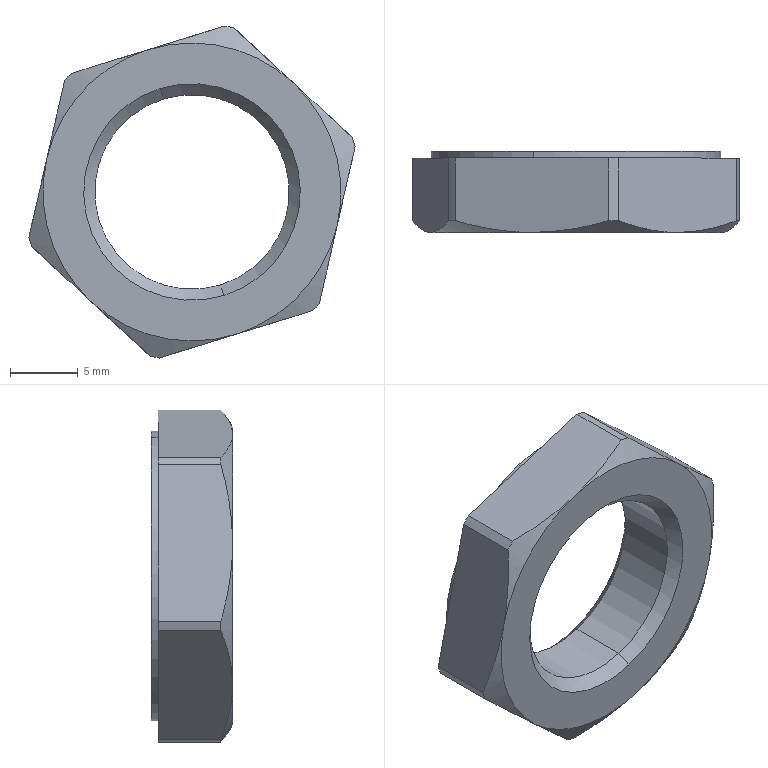Component | SolidWorks | gbgb16 MA NutF8-1 | 1 solid | 29 faces | box 24.09 x 6 x 24.52 mm | volume 1467 mm3 | cone 10 | cylinder 10 | plane 9 | commonest cylinder face diameters 25 x6 14.376 x2 21.4 x2
STEP:
#1=CARTESIAN_POINT('',(3.084,19.257,17.209));
#2=VERTEX_POINT('',#1);
#3=CARTESIAN_POINT('',(3.251,19.257,16.668));
#4=VERTEX_POINT('',#3);
#5=CARTESIAN_POINT('',(3.167,19.257,16.938));
#6=DIRECTION('',(0.,-1.,-0.));
#7=DIRECTION('',(0.2949,0.,-0.9555));
#8=AXIS2_PLACEMENT_3D('',#5,#6,#7);
#9=CIRCLE('',#8,0.283);
#10=EDGE_CURVE('',#2,#4,#9,.T.);
#11=ORIENTED_EDGE('',*,*,#10,.T.);
#12=CARTESIAN_POINT('',(3.26,19.289,16.637));
#13=VERTEX_POINT('',#12);
#14=CARTESIAN_POINT('',(3.26,19.289,16.637));
#15=DIRECTION('',(0.2085,0.7071,-0.6757));
#16=VECTOR('',#15,39.37);
#17=LINE('',#14,#16);
#18=EDGE_CURVE('',#4,#13,#17,.T.);
#19=ORIENTED_EDGE('',*,*,#18,.T.);
#20=CARTESIAN_POINT('',(3.074,19.289,17.239));
#21=VERTEX_POINT('',#20);
#22=CARTESIAN_POINT('',(3.167,19.289,16.938));
#23=DIRECTION('',(0.,-1.,-0.));
#24=DIRECTION('',(0.2949,0.,-0.9555));
#25=AXIS2_PLACEMENT_3D('',#22,#23,#24);
#26=CIRCLE('',#25,0.315);
#27=EDGE_CURVE('',#21,#13,#26,.T.);
#28=ORIENTED_EDGE('',*,*,#27,.F.);
#29=CARTESIAN_POINT('',(3.074,19.289,17.239));
#30=DIRECTION('',(-0.2085,0.7071,0.6757));
#31=VECTOR('',#30,39.37);
#32=LINE('',#29,#31);
#33=EDGE_CURVE('',#2,#21,#32,.T.);
#34=ORIENTED_EDGE('',*,*,#33,.F.);
#35=EDGE_LOOP('',(#11,#19,#28,#34));
#36=FACE_OUTER_BOUND('',#35,.T.);
#37=CARTESIAN_POINT('',(3.167,19.289,16.938));
#38=DIRECTION('',(-0.,1.,0.));
#39=DIRECTION('',(-0.2949,-0.,0.9555));
#40=AXIS2_PLACEMENT_3D('',#37,#38,#39);
#41=CONICAL_SURFACE('',#40,0.315,0.7854);
#42=ADVANCED_FACE('',(#36),#41,.F.);
#43=ORIENTED_EDGE('',*,*,#10,.F.);
#44=CARTESIAN_POINT('',(3.084,19.085,17.209));
#45=VERTEX_POINT('',#44);
#46=CARTESIAN_POINT('',(3.084,19.289,17.209));
#47=DIRECTION('',(0.,-1.,-0.));
#48=VECTOR('',#47,39.37);
#49=LINE('',#46,#48);
#50=EDGE_CURVE('',#2,#45,#49,.T.);
#51=ORIENTED_EDGE('',*,*,#50,.T.);
#52=CARTESIAN_POINT('',(3.251,19.085,16.668));
#53=VERTEX_POINT('',#52);
#54=CARTESIAN_POINT('',(3.167,19.085,16.938));
#55=DIRECTION('',(0.,-1.,-0.));
#56=DIRECTION('',(0.2949,0.,-0.9555));
#57=AXIS2_PLACEMENT_3D('',#54,#55,#56);
#58=CIRCLE('',#57,0.283);
#59=EDGE_CURVE('',#45,#53,#58,.T.);
#60=ORIENTED_EDGE('',*,*,#59,.T.);
#61=CARTESIAN_POINT('',(3.251,19.289,16.668));
#62=DIRECTION('',(0.,-1.,-0.));
#63=VECTOR('',#62,39.37);
#64=LINE('',#61,#63);
#65=EDGE_CURVE('',#4,#53,#64,.T.);
#66=ORIENTED_EDGE('',*,*,#65,.F.);
#67=EDGE_LOOP('',(#43,#51,#60,#66));
#68=FACE_OUTER_BOUND('',#67,.T.);
#69=CARTESIAN_POINT('',(3.167,19.289,16.938));
#70=DIRECTION('',(0.,-1.,-0.));
#71=DIRECTION('',(0.2949,0.,-0.9555));
#72=AXIS2_PLACEMENT_3D('',#69,#70,#71);
#73=CYLINDRICAL_SURFACE('',#72,0.283);
#74=ADVANCED_FACE('',(#68),#73,.F.);
#75=ORIENTED_EDGE('',*,*,#59,.F.);
#76=CARTESIAN_POINT('',(3.074,19.053,17.239));
#77=VERTEX_POINT('',#76);
#78=CARTESIAN_POINT('',(3.084,19.085,17.209));
#79=DIRECTION('',(-0.2085,-0.7071,0.6757));
#80=VECTOR('',#79,39.37);
#81=LINE('',#78,#80);
#82=EDGE_CURVE('',#45,#77,#81,.T.);
#83=ORIENTED_EDGE('',*,*,#82,.T.);
#84=CARTESIAN_POINT('',(3.26,19.053,16.637));
#85=VERTEX_POINT('',#84);
#86=CARTESIAN_POINT('',(3.167,19.053,16.938));
#87=DIRECTION('',(0.,-1.,-0.));
#88=DIRECTION('',(0.2949,0.,-0.9555));
#89=AXIS2_PLACEMENT_3D('',#86,#87,#88);
#90=CIRCLE('',#89,0.315);
#91=EDGE_CURVE('',#77,#85,#90,.T.);
#92=ORIENTED_EDGE('',*,*,#91,.T.);
#93=CARTESIAN_POINT('',(3.251,19.085,16.668));
#94=DIRECTION('',(0.2085,-0.7071,-0.6757));
#95=VECTOR('',#94,39.37);
#96=LINE('',#93,#95);
#97=EDGE_CURVE('',#53,#85,#96,.T.);
#98=ORIENTED_EDGE('',*,*,#97,.F.);
#99=EDGE_LOOP('',(#75,#83,#92,#98));
#100=FACE_OUTER_BOUND('',#99,.T.);
#101=CARTESIAN_POINT('',(3.167,19.085,16.938));
#102=DIRECTION('',(0.,-1.,-0.));
#103=DIRECTION('',(0.2949,0.,-0.9555));
#104=AXIS2_PLACEMENT_3D('',#101,#102,#103);
#105=CONICAL_SURFACE('',#104,0.283,0.7854);
#106=ADVANCED_FACE('',(#100),#105,.F.);
#107=CARTESIAN_POINT('',(3.291,19.289,16.536));
#108=VERTEX_POINT('',#107);
#109=CARTESIAN_POINT('',(3.043,19.289,17.341));
#110=VERTEX_POINT('',#109);
#111=CARTESIAN_POINT('',(3.167,19.289,16.938));
#112=DIRECTION('',(0.,-1.,-0.));
#113=DIRECTION('',(0.2949,0.,-0.9555));
#114=AXIS2_PLACEMENT_3D('',#111,#112,#113);
#115=CIRCLE('',#114,0.4213);
#116=EDGE_CURVE('',#108,#110,#115,.T.);
#117=ORIENTED_EDGE('',*,*,#116,.T.);
#118=CARTESIAN_POINT('',(3.043,19.269,17.341));
#119=VERTEX_POINT('',#118);
#120=CARTESIAN_POINT('',(3.043,19.289,17.341));
#121=DIRECTION('',(0.,-1.,-0.));
#122=VECTOR('',#121,39.37);
#123=LINE('',#120,#122);
#124=EDGE_CURVE('',#110,#119,#123,.T.);
#125=ORIENTED_EDGE('',*,*,#124,.T.);
#126=CARTESIAN_POINT('',(3.291,19.269,16.536));
#127=VERTEX_POINT('',#126);
#128=CARTESIAN_POINT('',(3.167,19.269,16.938));
#129=DIRECTION('',(0.,-1.,-0.));
#130=DIRECTION('',(0.2949,0.,-0.9555));
#131=AXIS2_PLACEMENT_3D('',#128,#129,#130);
#132=CIRCLE('',#131,0.4213);
#133=EDGE_CURVE('',#127,#119,#132,.T.);
#134=ORIENTED_EDGE('',*,*,#133,.F.);
#135=CARTESIAN_POINT('',(3.291,19.289,16.536));
#136=DIRECTION('',(0.,-1.,-0.));
#137=VECTOR('',#136,39.37);
#138=LINE('',#135,#137);
#139=EDGE_CURVE('',#108,#127,#138,.T.);
#140=ORIENTED_EDGE('',*,*,#139,.F.);
#141=EDGE_LOOP('',(#117,#125,#134,#140));
#142=FACE_OUTER_BOUND('',#141,.T.);
#143=CARTESIAN_POINT('',(3.167,19.289,16.938));
#144=DIRECTION('',(0.,-1.,-0.));
#145=DIRECTION('',(0.2949,0.,-0.9555));
#146=AXIS2_PLACEMENT_3D('',#143,#144,#145);
#147=CYLINDRICAL_SURFACE('',#146,0.4213);
#148=ADVANCED_FACE('',(#142),#147,.T.);
#149=CARTESIAN_POINT('',(3.518,19.087,16.593));
#150=VERTEX_POINT('',#149);
#151=CARTESIAN_POINT('',(3.537,19.087,16.614));
#152=VERTEX_POINT('',#151);
#153=CARTESIAN_POINT('',(3.167,19.087,16.938));
#154=DIRECTION('',(0.,-1.,-0.));
#155=DIRECTION('',(0.2949,0.,-0.9555));
#156=AXIS2_PLACEMENT_3D('',#153,#154,#155);
#157=CIRCLE('',#156,0.4921);
#158=EDGE_CURVE('',#150,#152,#157,.T.);
#159=ORIENTED_EDGE('',*,*,#158,.T.);
#160=CARTESIAN_POINT('',(3.589,19.053,16.842));
#161=VERTEX_POINT('',#160);
#162=CARTESIAN_POINT('',(3.537,19.087,16.614));
#163=CARTESIAN_POINT('',(3.546,19.076,16.651));
#164=CARTESIAN_POINT('',(3.555,19.068,16.689));
#165=CARTESIAN_POINT('',(3.572,19.056,16.765));
#166=CARTESIAN_POINT('',(3.581,19.053,16.803));
#167=CARTESIAN_POINT('',(3.589,19.053,16.842));
#168=B_SPLINE_CURVE_WITH_KNOTS('',3,(#162,#163,#164,#165,#166,#167),.UNSPECIFIED.,.F.,.F.,(4,2,4),(0.00000075,0.003,0.006),.UNSPECIFIED.);
#169=EDGE_CURVE('',#152,#161,#168,.T.);
#170=ORIENTED_EDGE('',*,*,#169,.T.);
#171=CARTESIAN_POINT('',(3.295,19.053,16.524));
#172=VERTEX_POINT('',#171);
#173=CARTESIAN_POINT('',(3.167,19.053,16.938));
#174=DIRECTION('',(0.,-1.,-0.));
#175=DIRECTION('',(0.2949,0.,-0.9555));
#176=AXIS2_PLACEMENT_3D('',#173,#174,#175);
#177=CIRCLE('',#176,0.4331);
#178=EDGE_CURVE('',#172,#161,#177,.T.);
#179=ORIENTED_EDGE('',*,*,#178,.F.);
#180=CARTESIAN_POINT('',(3.295,19.053,16.524));
#181=CARTESIAN_POINT('',(3.314,19.053,16.53));
#182=CARTESIAN_POINT('',(3.333,19.054,16.536));
#183=CARTESIAN_POINT('',(3.371,19.057,16.548));
#184=CARTESIAN_POINT('',(3.389,19.059,16.554));
#185=CARTESIAN_POINT('',(3.445,19.068,16.571));
#186=CARTESIAN_POINT('',(3.482,19.076,16.582));
#187=CARTESIAN_POINT('',(3.518,19.087,16.593));
#188=B_SPLINE_CURVE_WITH_KNOTS('',3,(#180,#181,#182,#183,#184,#185,#186,#187),.UNSPECIFIED.,.F.,.F.,(4,2,2,4),(0.01774,0.01924,0.02074,0.02374),.UNSPECIFIED.);
#189=EDGE_CURVE('',#172,#150,#188,.T.);
#190=ORIENTED_EDGE('',*,*,#189,.T.);
#191=EDGE_LOOP('',(#159,#170,#179,#190));
#192=FACE_OUTER_BOUND('',#191,.T.);
#193=CARTESIAN_POINT('',(3.167,19.087,16.938));
#194=DIRECTION('',(-0.,1.,0.));
#195=DIRECTION('',(-0.2949,-0.,0.9555));
#196=AXIS2_PLACEMENT_3D('',#193,#194,#195);
#197=CONICAL_SURFACE('',#196,0.4921,1.047);
#198=ADVANCED_FACE('',(#192),#197,.T.);
#199=CARTESIAN_POINT('',(3.044,19.087,16.462));
#200=VERTEX_POINT('',#199);
#201=CARTESIAN_POINT('',(3.072,19.087,16.456));
#202=VERTEX_POINT('',#201);
#203=CARTESIAN_POINT('',(3.167,19.087,16.938));
#204=DIRECTION('',(0.,-1.,-0.));
#205=DIRECTION('',(0.2949,0.,-0.9555));
#206=AXIS2_PLACEMENT_3D('',#203,#204,#205);
#207=CIRCLE('',#206,0.4921);
#208=EDGE_CURVE('',#200,#202,#207,.T.);
#209=ORIENTED_EDGE('',*,*,#208,.T.);
#210=CARTESIAN_POINT('',(3.072,19.087,16.456));
#211=CARTESIAN_POINT('',(3.108,19.076,16.467));
#212=CARTESIAN_POINT('',(3.145,19.068,16.478));
#213=CARTESIAN_POINT('',(3.22,19.056,16.501));
#214=CARTESIAN_POINT('',(3.257,19.053,16.513));
#215=CARTESIAN_POINT('',(3.295,19.053,16.524));
#216=B_SPLINE_CURVE_WITH_KNOTS('',3,(#210,#211,#212,#213,#214,#215),.UNSPECIFIED.,.F.,.F.,(4,2,4),(0.01174,0.01474,0.01774),.UNSPECIFIED.);
#217=EDGE_CURVE('',#202,#172,#216,.T.);
#218=ORIENTED_EDGE('',*,*,#217,.T.);
#219=CARTESIAN_POINT('',(2.873,19.053,16.621));
#220=VERTEX_POINT('',#219);
#221=CARTESIAN_POINT('',(3.167,19.053,16.938));
#222=DIRECTION('',(0.,-1.,-0.));
#223=DIRECTION('',(0.2949,0.,-0.9555));
#224=AXIS2_PLACEMENT_3D('',#221,#222,#223);
#225=CIRCLE('',#224,0.4331);
#226=EDGE_CURVE('',#220,#172,#225,.T.);
#227=ORIENTED_EDGE('',*,*,#226,.F.);
#228=CARTESIAN_POINT('',(2.873,19.053,16.621));
#229=CARTESIAN_POINT('',(2.887,19.053,16.607));
#230=CARTESIAN_POINT('',(2.902,19.054,16.594));
#231=CARTESIAN_POINT('',(2.931,19.057,16.567));
#232=CARTESIAN_POINT('',(2.945,19.059,16.554));
#233=CARTESIAN_POINT('',(2.988,19.068,16.514));
#234=CARTESIAN_POINT('',(3.016,19.076,16.488));
#235=CARTESIAN_POINT('',(3.044,19.087,16.462));
#236=B_SPLINE_CURVE_WITH_KNOTS('',3,(#228,#229,#230,#231,#232,#233,#234,#235),.UNSPECIFIED.,.F.,.F.,(4,2,2,4),(0.006,0.007491,0.008982,0.01196),.UNSPECIFIED.);
#237=EDGE_CURVE('',#220,#200,#236,.T.);
#238=ORIENTED_EDGE('',*,*,#237,.T.);
#239=EDGE_LOOP('',(#209,#218,#227,#238));
#240=FACE_OUTER_BOUND('',#239,.T.);
#241=CARTESIAN_POINT('',(3.167,19.087,16.938));
#242=DIRECTION('',(-0.,1.,0.));
#243=DIRECTION('',(-0.2949,-0.,0.9555));
#244=AXIS2_PLACEMENT_3D('',#241,#242,#243);
#245=CONICAL_SURFACE('',#244,0.4921,1.047);
#246=ADVANCED_FACE('',(#240),#245,.T.);
#247=CARTESIAN_POINT('',(2.693,19.087,16.807));
#248=VERTEX_POINT('',#247);
#249=CARTESIAN_POINT('',(2.701,19.087,16.78));
#250=VERTEX_POINT('',#249);
#251=CARTESIAN_POINT('',(3.167,19.087,16.938));
#252=DIRECTION('',(0.,-1.,-0.));
#253=DIRECTION('',(0.2949,0.,-0.9555));
#254=AXIS2_PLACEMENT_3D('',#251,#252,#253);
#255=CIRCLE('',#254,0.4921);
#256=EDGE_CURVE('',#248,#250,#255,.T.);
#257=ORIENTED_EDGE('',*,*,#256,.T.);
#258=CARTESIAN_POINT('',(2.701,19.087,16.78));
#259=CARTESIAN_POINT('',(2.729,19.076,16.754));
#260=CARTESIAN_POINT('',(2.758,19.068,16.727));
#261=CARTESIAN_POINT('',(2.815,19.056,16.674));
#262=CARTESIAN_POINT('',(2.844,19.053,16.648));
#263=CARTESIAN_POINT('',(2.873,19.053,16.621));
#264=B_SPLINE_CURVE_WITH_KNOTS('',3,(#258,#259,#260,#261,#262,#263),.UNSPECIFIED.,.F.,.F.,(4,2,4),(0.00000075,0.003,0.006),.UNSPECIFIED.);
#265=EDGE_CURVE('',#250,#220,#264,.T.);
#266=ORIENTED_EDGE('',*,*,#265,.T.);
#267=CARTESIAN_POINT('',(2.745,19.053,17.035));
#268=VERTEX_POINT('',#267);
#269=CARTESIAN_POINT('',(3.167,19.053,16.938));
#270=DIRECTION('',(0.,-1.,-0.));
#271=DIRECTION('',(0.2949,0.,-0.9555));
#272=AXIS2_PLACEMENT_3D('',#269,#270,#271);
#273=CIRCLE('',#272,0.4331);
#274=EDGE_CURVE('',#268,#220,#273,.T.);
#275=ORIENTED_EDGE('',*,*,#274,.F.);
#276=CARTESIAN_POINT('',(2.745,19.053,17.035));
#277=CARTESIAN_POINT('',(2.741,19.053,17.015));
#278=CARTESIAN_POINT('',(2.736,19.054,16.996));
#279=CARTESIAN_POINT('',(2.727,19.057,16.957));
#280=CARTESIAN_POINT('',(2.723,19.059,16.938));
#281=CARTESIAN_POINT('',(2.71,19.068,16.881));
#282=CARTESIAN_POINT('',(2.701,19.076,16.844));
#283=CARTESIAN_POINT('',(2.693,19.087,16.807));
#284=B_SPLINE_CURVE_WITH_KNOTS('',3,(#276,#277,#278,#279,#280,#281,#282,#283),.UNSPECIFIED.,.F.,.F.,(4,2,2,4),(0.006,0.007491,0.008982,0.01196),.UNSPECIFIED.);
#285=EDGE_CURVE('',#268,#248,#284,.T.);
#286=ORIENTED_EDGE('',*,*,#285,.T.);
#287=EDGE_LOOP('',(#257,#266,#275,#286));
#288=FACE_OUTER_BOUND('',#287,.T.);
#289=CARTESIAN_POINT('',(3.167,19.087,16.938));
#290=DIRECTION('',(-0.,1.,0.));
#291=DIRECTION('',(-0.2949,-0.,0.9555));
#292=AXIS2_PLACEMENT_3D('',#289,#290,#291);
#293=CONICAL_SURFACE('',#292,0.4921,1.047);
#294=ADVANCED_FACE('',(#288),#293,.T.);
#295=CARTESIAN_POINT('',(2.816,19.087,17.283));
#296=VERTEX_POINT('',#295);
#297=CARTESIAN_POINT('',(2.797,19.087,17.262));
#298=VERTEX_POINT('',#297);
#299=CARTESIAN_POINT('',(3.167,19.087,16.938));
#300=DIRECTION('',(0.,-1.,-0.));
#301=DIRECTION('',(0.2949,0.,-0.9555));
#302=AXIS2_PLACEMENT_3D('',#299,#300,#301);
#303=CIRCLE('',#302,0.4921);
#304=EDGE_CURVE('',#296,#298,#303,.T.);
#305=ORIENTED_EDGE('',*,*,#304,.T.);
#306=CARTESIAN_POINT('',(2.797,19.087,17.262));
#307=CARTESIAN_POINT('',(2.788,19.076,17.225));
#308=CARTESIAN_POINT('',(2.78,19.068,17.187));
#309=CARTESIAN_POINT('',(2.762,19.056,17.112));
#310=CARTESIAN_POINT('',(2.754,19.053,17.073));
#311=CARTESIAN_POINT('',(2.745,19.053,17.035));
#312=B_SPLINE_CURVE_WITH_KNOTS('',3,(#306,#307,#308,#309,#310,#311),.UNSPECIFIED.,.F.,.F.,(4,2,4),(0.00000075,0.003,0.006),.UNSPECIFIED.);
#313=EDGE_CURVE('',#298,#268,#312,.T.);
#314=ORIENTED_EDGE('',*,*,#313,.T.);
#315=CARTESIAN_POINT('',(3.039,19.053,17.352));
#316=VERTEX_POINT('',#315);
#317=CARTESIAN_POINT('',(3.167,19.053,16.938));
#318=DIRECTION('',(0.,-1.,-0.));
#319=DIRECTION('',(0.2949,0.,-0.9555));
#320=AXIS2_PLACEMENT_3D('',#317,#318,#319);
#321=CIRCLE('',#320,0.4331);
#322=EDGE_CURVE('',#316,#268,#321,.T.);
#323=ORIENTED_EDGE('',*,*,#322,.F.);
#324=CARTESIAN_POINT('',(3.039,19.053,17.352));
#325=CARTESIAN_POINT('',(3.002,19.053,17.34));
#326=CARTESIAN_POINT('',(2.964,19.056,17.329));
#327=CARTESIAN_POINT('',(2.89,19.068,17.306));
#328=CARTESIAN_POINT('',(2.853,19.076,17.294));
#329=CARTESIAN_POINT('',(2.816,19.087,17.283));
#330=B_SPLINE_CURVE_WITH_KNOTS('',3,(#324,#325,#326,#327,#328,#329),.UNSPECIFIED.,.F.,.F.,(4,2,4),(0.01109,0.01408,0.01707),.UNSPECIFIED.);
#331=EDGE_CURVE('',#316,#296,#330,.T.);
#332=ORIENTED_EDGE('',*,*,#331,.T.);
#333=EDGE_LOOP('',(#305,#314,#323,#332));
#334=FACE_OUTER_BOUND('',#333,.T.);
#335=CARTESIAN_POINT('',(3.167,19.087,16.938));
#336=DIRECTION('',(-0.,1.,0.));
#337=DIRECTION('',(-0.2949,-0.,0.9555));
#338=AXIS2_PLACEMENT_3D('',#335,#336,#337);
#339=CONICAL_SURFACE('',#338,0.4921,1.047);
#340=ADVANCED_FACE('',(#334),#339,.T.);
#341=CARTESIAN_POINT('',(3.29,19.087,17.415));
#342=VERTEX_POINT('',#341);
#343=CARTESIAN_POINT('',(3.263,19.087,17.421));
#344=VERTEX_POINT('',#343);
#345=CARTESIAN_POINT('',(3.167,19.087,16.938));
#346=DIRECTION('',(0.,-1.,-0.));
#347=DIRECTION('',(0.2949,0.,-0.9555));
#348=AXIS2_PLACEMENT_3D('',#345,#346,#347);
#349=CIRCLE('',#348,0.4921);
#350=EDGE_CURVE('',#342,#344,#349,.T.);
#351=ORIENTED_EDGE('',*,*,#350,.T.);
#352=CARTESIAN_POINT('',(3.263,19.087,17.421));
#353=CARTESIAN_POINT('',(3.227,19.076,17.41));
#354=CARTESIAN_POINT('',(3.19,19.068,17.399));
#355=CARTESIAN_POINT('',(3.134,19.059,17.381));
#356=CARTESIAN_POINT('',(3.115,19.057,17.375));
#357=CARTESIAN_POINT('',(3.077,19.054,17.364));
#358=CARTESIAN_POINT('',(3.058,19.053,17.358));
#359=CARTESIAN_POINT('',(3.039,19.053,17.352));
#360=B_SPLINE_CURVE_WITH_KNOTS('',3,(#352,#353,#354,#355,#356,#357,#358,#359),.UNSPECIFIED.,.F.,.F.,(4,2,2,4),(0.005104,0.008096,0.009591,0.01109),.UNSPECIFIED.);
#361=EDGE_CURVE('',#344,#316,#360,.T.);
#362=ORIENTED_EDGE('',*,*,#361,.T.);
#363=CARTESIAN_POINT('',(3.462,19.053,17.256));
#364=VERTEX_POINT('',#363);
#365=CARTESIAN_POINT('',(3.167,19.053,16.938));
#366=DIRECTION('',(0.,-1.,-0.));
#367=DIRECTION('',(0.2949,0.,-0.9555));
#368=AXIS2_PLACEMENT_3D('',#365,#366,#367);
#369=CIRCLE('',#368,0.4331);
#370=EDGE_CURVE('',#364,#316,#369,.T.);
#371=ORIENTED_EDGE('',*,*,#370,.F.);
#372=CARTESIAN_POINT('',(3.462,19.053,17.256));
#373=CARTESIAN_POINT('',(3.447,19.053,17.269));
#374=CARTESIAN_POINT('',(3.433,19.054,17.283));
#375=CARTESIAN_POINT('',(3.404,19.057,17.31));
#376=CARTESIAN_POINT('',(3.389,19.059,17.323));
#377=CARTESIAN_POINT('',(3.347,19.068,17.363));
#378=CARTESIAN_POINT('',(3.318,19.076,17.389));
#379=CARTESIAN_POINT('',(3.29,19.087,17.415));
#380=B_SPLINE_CURVE_WITH_KNOTS('',3,(#372,#373,#374,#375,#376,#377,#378,#379),.UNSPECIFIED.,.F.,.F.,(4,2,2,4),(0.006,0.007491,0.008982,0.01196),.UNSPECIFIED.);
#381=EDGE_CURVE('',#364,#342,#380,.T.);
#382=ORIENTED_EDGE('',*,*,#381,.T.);
#383=EDGE_LOOP('',(#351,#362,#371,#382));
#384=FACE_OUTER_BOUND('',#383,.T.);
#385=CARTESIAN_POINT('',(3.167,19.087,16.938));
#386=DIRECTION('',(-0.,1.,0.));
#387=DIRECTION('',(-0.2949,-0.,0.9555));
#388=AXIS2_PLACEMENT_3D('',#385,#386,#387);
#389=CONICAL_SURFACE('',#388,0.4921,1.047);
#390=ADVANCED_FACE('',(#384),#389,.T.);
#391=CARTESIAN_POINT('',(3.518,19.269,16.593));
#392=VERTEX_POINT('',#391);
#393=CARTESIAN_POINT('',(3.537,19.269,16.614));
#394=VERTEX_POINT('',#393);
#395=CARTESIAN_POINT('',(3.167,19.269,16.938));
#396=DIRECTION('',(0.,-1.,-0.));
#397=DIRECTION('',(0.2949,0.,-0.9555));
#398=AXIS2_PLACEMENT_3D('',#395,#396,#397);
#399=CIRCLE('',#398,0.4921);
#400=EDGE_CURVE('',#392,#394,#399,.T.);
#401=ORIENTED_EDGE('',*,*,#400,.T.);
#402=CARTESIAN_POINT('',(3.537,19.289,16.614));
#403=DIRECTION('',(0.,-1.,-0.));
#404=VECTOR('',#403,39.37);
#405=LINE('',#402,#404);
#406=EDGE_CURVE('',#394,#152,#405,.T.);
#407=ORIENTED_EDGE('',*,*,#406,.T.);
#408=ORIENTED_EDGE('',*,*,#158,.F.);
#409=CARTESIAN_POINT('',(3.518,19.289,16.593));
#410=DIRECTION('',(-0.,1.,0.));
#411=VECTOR('',#410,39.37);
#412=LINE('',#409,#411);
#413=EDGE_CURVE('',#150,#392,#412,.T.);
#414=ORIENTED_EDGE('',*,*,#413,.T.);
#415=EDGE_LOOP('',(#401,#407,#408,#414));
#416=FACE_OUTER_BOUND('',#415,.T.);
#417=CARTESIAN_POINT('',(3.167,19.289,16.938));
#418=DIRECTION('',(0.,-1.,-0.));
#419=DIRECTION('',(0.2949,0.,-0.9555));
#420=AXIS2_PLACEMENT_3D('',#417,#418,#419);
#421=CYLINDRICAL_SURFACE('',#420,0.4921);
#422=ADVANCED_FACE('',(#416),#421,.T.);
#423=CARTESIAN_POINT('',(3.044,19.269,16.462));
#424=VERTEX_POINT('',#423);
#425=CARTESIAN_POINT('',(3.072,19.269,16.456));
#426=VERTEX_POINT('',#425);
#427=CARTESIAN_POINT('',(3.167,19.269,16.938));
#428=DIRECTION('',(0.,-1.,-0.));
#429=DIRECTION('',(0.2949,0.,-0.9555));
#430=AXIS2_PLACEMENT_3D('',#427,#428,#429);
#431=CIRCLE('',#430,0.4921);
#432=EDGE_CURVE('',#424,#426,#431,.T.);
#433=ORIENTED_EDGE('',*,*,#432,.T.);
#434=CARTESIAN_POINT('',(3.072,19.289,16.456));
#435=DIRECTION('',(0.,-1.,-0.));
#436=VECTOR('',#435,39.37);
#437=LINE('',#434,#436);
#438=EDGE_CURVE('',#426,#202,#437,.T.);
#439=ORIENTED_EDGE('',*,*,#438,.T.);
#440=ORIENTED_EDGE('',*,*,#208,.F.);
#441=CARTESIAN_POINT('',(3.044,19.289,16.462));
#442=DIRECTION('',(-0.,1.,0.));
#443=VECTOR('',#442,39.37);
#444=LINE('',#441,#443);
#445=EDGE_CURVE('',#200,#424,#444,.T.);
#446=ORIENTED_EDGE('',*,*,#445,.T.);
#447=EDGE_LOOP('',(#433,#439,#440,#446));
#448=FACE_OUTER_BOUND('',#447,.T.);
#449=CARTESIAN_POINT('',(3.167,19.289,16.938));
#450=DIRECTION('',(0.,-1.,-0.));
#451=DIRECTION('',(0.2949,0.,-0.9555));
#452=AXIS2_PLACEMENT_3D('',#449,#450,#451);
#453=CYLINDRICAL_SURFACE('',#452,0.4921);
#454=ADVANCED_FACE('',(#448),#453,.T.);
#455=CARTESIAN_POINT('',(2.693,19.269,16.807));
#456=VERTEX_POINT('',#455);
#457=CARTESIAN_POINT('',(2.701,19.269,16.78));
#458=VERTEX_POINT('',#457);
#459=CARTESIAN_POINT('',(3.167,19.269,16.938));
#460=DIRECTION('',(0.,-1.,-0.));
#461=DIRECTION('',(0.2949,0.,-0.9555));
#462=AXIS2_PLACEMENT_3D('',#459,#460,#461);
#463=CIRCLE('',#462,0.4921);
#464=EDGE_CURVE('',#456,#458,#463,.T.);
#465=ORIENTED_EDGE('',*,*,#464,.T.);
#466=CARTESIAN_POINT('',(2.701,19.289,16.78));
#467=DIRECTION('',(0.,-1.,-0.));
#468=VECTOR('',#467,39.37);
#469=LINE('',#466,#468);
#470=EDGE_CURVE('',#458,#250,#469,.T.);
#471=ORIENTED_EDGE('',*,*,#470,.T.);
#472=ORIENTED_EDGE('',*,*,#256,.F.);
#473=CARTESIAN_POINT('',(2.693,19.289,16.807));
#474=DIRECTION('',(-0.,1.,0.));
#475=VECTOR('',#474,39.37);
#476=LINE('',#473,#475);
#477=EDGE_CURVE('',#248,#456,#476,.T.);
#478=ORIENTED_EDGE('',*,*,#477,.T.);
#479=EDGE_LOOP('',(#465,#471,#472,#478));
#480=FACE_OUTER_BOUND('',#479,.T.);
#481=CARTESIAN_POINT('',(3.167,19.289,16.938));
#482=DIRECTION('',(0.,-1.,-0.));
#483=DIRECTION('',(0.2949,0.,-0.9555));
#484=AXIS2_PLACEMENT_3D('',#481,#482,#483);
#485=CYLINDRICAL_SURFACE('',#484,0.4921);
#486=ADVANCED_FACE('',(#480),#485,.T.);
#487=CARTESIAN_POINT('',(2.816,19.269,17.283));
#488=VERTEX_POINT('',#487);
#489=CARTESIAN_POINT('',(2.797,19.269,17.262));
#490=VERTEX_POINT('',#489);
#491=CARTESIAN_POINT('',(3.167,19.269,16.938));
#492=DIRECTION('',(0.,-1.,-0.));
#493=DIRECTION('',(0.2949,0.,-0.9555));
#494=AXIS2_PLACEMENT_3D('',#491,#492,#493);
#495=CIRCLE('',#494,0.4921);
#496=EDGE_CURVE('',#488,#490,#495,.T.);
#497=ORIENTED_EDGE('',*,*,#496,.T.);
#498=CARTESIAN_POINT('',(2.797,19.289,17.262));
#499=DIRECTION('',(0.,-1.,-0.));
#500=VECTOR('',#499,39.37);
#501=LINE('',#498,#500);
#502=EDGE_CURVE('',#490,#298,#501,.T.);
#503=ORIENTED_EDGE('',*,*,#502,.T.);
#504=ORIENTED_EDGE('',*,*,#304,.F.);
#505=CARTESIAN_POINT('',(2.816,19.289,17.283));
#506=DIRECTION('',(-0.,1.,0.));
#507=VECTOR('',#506,39.37);
#508=LINE('',#505,#507);
#509=EDGE_CURVE('',#296,#488,#508,.T.);
#510=ORIENTED_EDGE('',*,*,#509,.T.);
#511=EDGE_LOOP('',(#497,#503,#504,#510));
#512=FACE_OUTER_BOUND('',#511,.T.);
#513=CARTESIAN_POINT('',(3.167,19.289,16.938));
#514=DIRECTION('',(0.,-1.,-0.));
#515=DIRECTION('',(0.2949,0.,-0.9555));
#516=AXIS2_PLACEMENT_3D('',#513,#514,#515);
#517=CYLINDRICAL_SURFACE('',#516,0.4921);
#518=ADVANCED_FACE('',(#512),#517,.T.);
#519=CARTESIAN_POINT('',(3.29,19.269,17.415));
#520=VERTEX_POINT('',#519);
#521=CARTESIAN_POINT('',(3.263,19.269,17.421));
#522=VERTEX_POINT('',#521);
#523=CARTESIAN_POINT('',(3.167,19.269,16.938));
#524=DIRECTION('',(0.,-1.,-0.));
#525=DIRECTION('',(0.2949,0.,-0.9555));
#526=AXIS2_PLACEMENT_3D('',#523,#524,#525);
#527=CIRCLE('',#526,0.4921);
#528=EDGE_CURVE('',#520,#522,#527,.T.);
#529=ORIENTED_EDGE('',*,*,#528,.T.);
#530=CARTESIAN_POINT('',(3.263,19.289,17.421));
#531=DIRECTION('',(0.,-1.,-0.));
#532=VECTOR('',#531,39.37);
#533=LINE('',#530,#532);
#534=EDGE_CURVE('',#522,#344,#533,.T.);
#535=ORIENTED_EDGE('',*,*,#534,.T.);
#536=ORIENTED_EDGE('',*,*,#350,.F.);
#537=CARTESIAN_POINT('',(3.29,19.289,17.415));
#538=DIRECTION('',(-0.,1.,0.));
#539=VECTOR('',#538,39.37);
#540=LINE('',#537,#539);
#541=EDGE_CURVE('',#342,#520,#540,.T.);
#542=ORIENTED_EDGE('',*,*,#541,.T.);
#543=EDGE_LOOP('',(#529,#535,#536,#542));
#544=FACE_OUTER_BOUND('',#543,.T.);
#545=CARTESIAN_POINT('',(3.167,19.289,16.938));
#546=DIRECTION('',(0.,-1.,-0.));
#547=DIRECTION('',(0.2949,0.,-0.9555));
#548=AXIS2_PLACEMENT_3D('',#545,#546,#547);
#549=CYLINDRICAL_SURFACE('',#548,0.4921);
#550=ADVANCED_FACE('',(#544),#549,.T.);
#551=ORIENTED_EDGE('',*,*,#178,.T.);
#552=CARTESIAN_POINT('',(3.167,19.053,16.938));
#553=DIRECTION('',(0.,-1.,-0.));
#554=DIRECTION('',(0.2949,0.,-0.9555));
#555=AXIS2_PLACEMENT_3D('',#552,#553,#554);
#556=CIRCLE('',#555,0.4331);
#557=EDGE_CURVE('',#161,#364,#556,.T.);
#558=ORIENTED_EDGE('',*,*,#557,.T.);
#559=ORIENTED_EDGE('',*,*,#370,.T.);
#560=ORIENTED_EDGE('',*,*,#322,.T.);
#561=ORIENTED_EDGE('',*,*,#274,.T.);
#562=ORIENTED_EDGE('',*,*,#226,.T.);
#563=EDGE_LOOP('',(#551,#558,#559,#560,#561,#562));
#564=FACE_OUTER_BOUND('',#563,.T.);
#565=CARTESIAN_POINT('',(3.167,19.053,16.938));
#566=DIRECTION('',(0.,-1.,-0.));
#567=DIRECTION('',(0.2949,0.,-0.9555));
#568=AXIS2_PLACEMENT_3D('',#565,#566,#567);
#569=CIRCLE('',#568,0.315);
#570=EDGE_CURVE('',#85,#77,#569,.T.);
#571=ORIENTED_EDGE('',*,*,#570,.F.);
#572=ORIENTED_EDGE('',*,*,#91,.F.);
#573=EDGE_LOOP('',(#571,#572));
#574=FACE_BOUND('',#573,.T.);
#575=CARTESIAN_POINT('',(3.167,19.053,16.938));
#576=DIRECTION('',(-0.,1.,0.));
#577=DIRECTION('',(-0.2949,-0.,0.9555));
#578=AXIS2_PLACEMENT_3D('',#575,#576,#577);
#579=PLANE('',#578);
#580=ADVANCED_FACE('',(#564,#574),#579,.F.);
#581=ORIENTED_EDGE('',*,*,#116,.F.);
#582=CARTESIAN_POINT('',(3.167,19.289,16.938));
#583=DIRECTION('',(0.,-1.,-0.));
#584=DIRECTION('',(0.2949,0.,-0.9555));
#585=AXIS2_PLACEMENT_3D('',#582,#583,#584);
#586=CIRCLE('',#585,0.4213);
#587=EDGE_CURVE('',#110,#108,#586,.T.);
#588=ORIENTED_EDGE('',*,*,#587,.F.);
#589=EDGE_LOOP('',(#581,#588));
#590=FACE_OUTER_BOUND('',#589,.T.);
#591=ORIENTED_EDGE('',*,*,#27,.T.);
#592=CARTESIAN_POINT('',(3.167,19.289,16.938));
#593=DIRECTION('',(0.,-1.,-0.));
#594=DIRECTION('',(0.2949,0.,-0.9555));
#595=AXIS2_PLACEMENT_3D('',#592,#593,#594);
#596=CIRCLE('',#595,0.315);
#597=EDGE_CURVE('',#13,#21,#596,.T.);
#598=ORIENTED_EDGE('',*,*,#597,.T.);
#599=EDGE_LOOP('',(#591,#598));
#600=FACE_BOUND('',#599,.T.);
#601=CARTESIAN_POINT('',(3.57,19.289,17.062));
#602=DIRECTION('',(0.,-1.,-0.));
#603=DIRECTION('',(0.2949,0.,-0.9555));
#604=AXIS2_PLACEMENT_3D('',#601,#602,#603);
#605=PLANE('',#604);
#606=ADVANCED_FACE('',(#590,#600),#605,.F.);
#607=ORIENTED_EDGE('',*,*,#557,.F.);
#608=CARTESIAN_POINT('',(3.641,19.087,17.07));
#609=VERTEX_POINT('',#608);
#610=CARTESIAN_POINT('',(3.589,19.053,16.842));
#611=CARTESIAN_POINT('',(3.594,19.053,16.861));
#612=CARTESIAN_POINT('',(3.598,19.054,16.881));
#613=CARTESIAN_POINT('',(3.607,19.057,16.919));
#614=CARTESIAN_POINT('',(3.611,19.059,16.938));
#615=CARTESIAN_POINT('',(3.624,19.068,16.995));
#616=CARTESIAN_POINT('',(3.633,19.076,17.033));
#617=CARTESIAN_POINT('',(3.641,19.087,17.07));
#618=B_SPLINE_CURVE_WITH_KNOTS('',3,(#610,#611,#612,#613,#614,#615,#616,#617),.UNSPECIFIED.,.F.,.F.,(4,2,2,4),(0.006,0.007491,0.008982,0.01196),.UNSPECIFIED.);
#619=EDGE_CURVE('',#161,#609,#618,.T.);
#620=ORIENTED_EDGE('',*,*,#619,.T.);
#621=CARTESIAN_POINT('',(3.633,19.087,17.097));
#622=VERTEX_POINT('',#621);
#623=CARTESIAN_POINT('',(3.167,19.087,16.938));
#624=DIRECTION('',(0.,-1.,-0.));
#625=DIRECTION('',(0.2949,0.,-0.9555));
#626=AXIS2_PLACEMENT_3D('',#623,#624,#625);
#627=CIRCLE('',#626,0.4921);
#628=EDGE_CURVE('',#609,#622,#627,.T.);
#629=ORIENTED_EDGE('',*,*,#628,.T.);
#630=CARTESIAN_POINT('',(3.633,19.087,17.097));
#631=CARTESIAN_POINT('',(3.605,19.076,17.123));
#632=CARTESIAN_POINT('',(3.577,19.068,17.149));
#633=CARTESIAN_POINT('',(3.52,19.056,17.202));
#634=CARTESIAN_POINT('',(3.491,19.053,17.229));
#635=CARTESIAN_POINT('',(3.462,19.053,17.256));
#636=B_SPLINE_CURVE_WITH_KNOTS('',3,(#630,#631,#632,#633,#634,#635),.UNSPECIFIED.,.F.,.F.,(4,2,4),(0.00000075,0.003,0.006),.UNSPECIFIED.);
#637=EDGE_CURVE('',#622,#364,#636,.T.);
#638=ORIENTED_EDGE('',*,*,#637,.T.);
#639=EDGE_LOOP('',(#607,#620,#629,#638));
#640=FACE_OUTER_BOUND('',#639,.T.);
#641=CARTESIAN_POINT('',(3.167,19.087,16.938));
#642=DIRECTION('',(-0.,1.,0.));
#643=DIRECTION('',(-0.2949,-0.,0.9555));
#644=AXIS2_PLACEMENT_3D('',#641,#642,#643);
#645=CONICAL_SURFACE('',#644,0.4921,1.047);
#646=ADVANCED_FACE('',(#640),#645,.T.);
#647=ORIENTED_EDGE('',*,*,#628,.F.);
#648=CARTESIAN_POINT('',(3.641,19.269,17.07));
#649=VERTEX_POINT('',#648);
#650=CARTESIAN_POINT('',(3.641,19.289,17.07));
#651=DIRECTION('',(-0.,1.,0.));
#652=VECTOR('',#651,39.37);
#653=LINE('',#650,#652);
#654=EDGE_CURVE('',#609,#649,#653,.T.);
#655=ORIENTED_EDGE('',*,*,#654,.T.);
#656=CARTESIAN_POINT('',(3.633,19.269,17.097));
#657=VERTEX_POINT('',#656);
#658=CARTESIAN_POINT('',(3.167,19.269,16.938));
#659=DIRECTION('',(0.,-1.,-0.));
#660=DIRECTION('',(0.2949,0.,-0.9555));
#661=AXIS2_PLACEMENT_3D('',#658,#659,#660);
#662=CIRCLE('',#661,0.4921);
#663=EDGE_CURVE('',#649,#657,#662,.T.);
#664=ORIENTED_EDGE('',*,*,#663,.T.);
#665=CARTESIAN_POINT('',(3.633,19.289,17.097));
#666=DIRECTION('',(0.,-1.,-0.));
#667=VECTOR('',#666,39.37);
#668=LINE('',#665,#667);
#669=EDGE_CURVE('',#657,#622,#668,.T.);
#670=ORIENTED_EDGE('',*,*,#669,.T.);
#671=EDGE_LOOP('',(#647,#655,#664,#670));
#672=FACE_OUTER_BOUND('',#671,.T.);
#673=CARTESIAN_POINT('',(3.167,19.289,16.938));
#674=DIRECTION('',(0.,-1.,-0.));
#675=DIRECTION('',(0.2949,0.,-0.9555));
#676=AXIS2_PLACEMENT_3D('',#673,#674,#675);
#677=CYLINDRICAL_SURFACE('',#676,0.4921);
#678=ADVANCED_FACE('',(#672),#677,.T.);
#679=ORIENTED_EDGE('',*,*,#663,.F.);
#680=CARTESIAN_POINT('',(3.644,19.269,17.082));
#681=DIRECTION('',(-0.2223,-0.,-0.975));
#682=VECTOR('',#681,39.37);
#683=LINE('',#680,#682);
#684=EDGE_CURVE('',#649,#394,#683,.T.);
#685=ORIENTED_EDGE('',*,*,#684,.T.);
#686=ORIENTED_EDGE('',*,*,#400,.F.);
#687=CARTESIAN_POINT('',(3.765,19.269,16.67));
#688=DIRECTION('',(-0.9555,-0.,-0.2949));
#689=VECTOR('',#688,39.37);
#690=LINE('',#687,#689);
#691=EDGE_CURVE('',#392,#426,#690,.T.);
#692=ORIENTED_EDGE('',*,*,#691,.T.);
#693=ORIENTED_EDGE('',*,*,#432,.F.);
#694=CARTESIAN_POINT('',(3.053,19.269,16.453));
#695=DIRECTION('',(-0.7332,-0.,0.68));
#696=VECTOR('',#695,39.37);
#697=LINE('',#694,#696);
#698=EDGE_CURVE('',#424,#458,#697,.T.);
#699=ORIENTED_EDGE('',*,*,#698,.T.);
#700=ORIENTED_EDGE('',*,*,#464,.F.);
#701=CARTESIAN_POINT('',(2.8,19.269,17.274));
#702=DIRECTION('',(0.2223,0.,0.975));
#703=VECTOR('',#702,39.37);
#704=LINE('',#701,#703);
#705=EDGE_CURVE('',#456,#490,#704,.T.);
#706=ORIENTED_EDGE('',*,*,#705,.T.);
#707=ORIENTED_EDGE('',*,*,#496,.F.);
#708=CARTESIAN_POINT('',(3.51,19.269,17.497));
#709=DIRECTION('',(0.9555,0.,0.2949));
#710=VECTOR('',#709,39.37);
#711=LINE('',#708,#710);
#712=EDGE_CURVE('',#488,#522,#711,.T.);
#713=ORIENTED_EDGE('',*,*,#712,.T.);
#714=ORIENTED_EDGE('',*,*,#528,.F.);
#715=CARTESIAN_POINT('',(3.642,19.269,17.088));
#716=DIRECTION('',(0.7332,0.,-0.68));
#717=VECTOR('',#716,39.37);
#718=LINE('',#715,#717);
#719=EDGE_CURVE('',#520,#657,#718,.T.);
#720=ORIENTED_EDGE('',*,*,#719,.T.);
#721=EDGE_LOOP('',(#679,#685,#686,#692,#693,#699,#700,#706,#707,#713,#714,#720));
#722=FACE_OUTER_BOUND('',#721,.T.);
#723=ORIENTED_EDGE('',*,*,#133,.T.);
#724=CARTESIAN_POINT('',(3.167,19.269,16.938));
#725=DIRECTION('',(0.,-1.,-0.));
#726=DIRECTION('',(0.2949,0.,-0.9555));
#727=AXIS2_PLACEMENT_3D('',#724,#725,#726);
#728=CIRCLE('',#727,0.4213);
#729=EDGE_CURVE('',#119,#127,#728,.T.);
#730=ORIENTED_EDGE('',*,*,#729,.T.);
#731=EDGE_LOOP('',(#723,#730));
#732=FACE_BOUND('',#731,.T.);
#733=CARTESIAN_POINT('',(3.637,19.269,17.083));
#734=DIRECTION('',(0.,-1.,-0.));
#735=DIRECTION('',(0.2949,0.,-0.9555));
#736=AXIS2_PLACEMENT_3D('',#733,#734,#735);
#737=PLANE('',#736);
#738=ADVANCED_FACE('',(#722,#732),#737,.F.);
#739=ORIENTED_EDGE('',*,*,#124,.F.);
#740=ORIENTED_EDGE('',*,*,#587,.T.);
#741=ORIENTED_EDGE('',*,*,#139,.T.);
#742=ORIENTED_EDGE('',*,*,#729,.F.);
#743=EDGE_LOOP('',(#739,#740,#741,#742));
#744=FACE_OUTER_BOUND('',#743,.T.);
#745=CARTESIAN_POINT('',(3.167,19.289,16.938));
#746=DIRECTION('',(0.,-1.,-0.));
#747=DIRECTION('',(0.2949,0.,-0.9555));
#748=AXIS2_PLACEMENT_3D('',#745,#746,#747);
#749=CYLINDRICAL_SURFACE('',#748,0.4213);
#750=ADVANCED_FACE('',(#744),#749,.T.);
#751=ORIENTED_EDGE('',*,*,#82,.F.);
#752=CARTESIAN_POINT('',(3.167,19.085,16.938));
#753=DIRECTION('',(0.,-1.,-0.));
#754=DIRECTION('',(0.2949,0.,-0.9555));
#755=AXIS2_PLACEMENT_3D('',#752,#753,#754);
#756=CIRCLE('',#755,0.283);
#757=EDGE_CURVE('',#53,#45,#756,.T.);
#758=ORIENTED_EDGE('',*,*,#757,.F.);
#759=ORIENTED_EDGE('',*,*,#97,.T.);
#760=ORIENTED_EDGE('',*,*,#570,.T.);
#761=EDGE_LOOP('',(#751,#758,#759,#760));
#762=FACE_OUTER_BOUND('',#761,.T.);
#763=CARTESIAN_POINT('',(3.167,19.085,16.938));
#764=DIRECTION('',(0.,-1.,-0.));
#765=DIRECTION('',(0.2949,0.,-0.9555));
#766=AXIS2_PLACEMENT_3D('',#763,#764,#765);
#767=CONICAL_SURFACE('',#766,0.283,0.7854);
#768=ADVANCED_FACE('',(#762),#767,.F.);
#769=ORIENTED_EDGE('',*,*,#50,.F.);
#770=CARTESIAN_POINT('',(3.167,19.257,16.938));
#771=DIRECTION('',(0.,-1.,-0.));
#772=DIRECTION('',(0.2949,0.,-0.9555));
#773=AXIS2_PLACEMENT_3D('',#770,#771,#772);
#774=CIRCLE('',#773,0.283);
#775=EDGE_CURVE('',#4,#2,#774,.T.);
#776=ORIENTED_EDGE('',*,*,#775,.F.);
#777=ORIENTED_EDGE('',*,*,#65,.T.);
#778=ORIENTED_EDGE('',*,*,#757,.T.);
#779=EDGE_LOOP('',(#769,#776,#777,#778));
#780=FACE_OUTER_BOUND('',#779,.T.);
#781=CARTESIAN_POINT('',(3.167,19.289,16.938));
#782=DIRECTION('',(0.,-1.,-0.));
#783=DIRECTION('',(0.2949,0.,-0.9555));
#784=AXIS2_PLACEMENT_3D('',#781,#782,#783);
#785=CYLINDRICAL_SURFACE('',#784,0.283);
#786=ADVANCED_FACE('',(#780),#785,.F.);
#787=ORIENTED_EDGE('',*,*,#18,.F.);
#788=ORIENTED_EDGE('',*,*,#775,.T.);
#789=ORIENTED_EDGE('',*,*,#33,.T.);
#790=ORIENTED_EDGE('',*,*,#597,.F.);
#791=EDGE_LOOP('',(#787,#788,#789,#790));
#792=FACE_OUTER_BOUND('',#791,.T.);
#793=CARTESIAN_POINT('',(3.167,19.289,16.938));
#794=DIRECTION('',(-0.,1.,0.));
#795=DIRECTION('',(-0.2949,-0.,0.9555));
#796=AXIS2_PLACEMENT_3D('',#793,#794,#795);
#797=CONICAL_SURFACE('',#796,0.315,0.7854);
#798=ADVANCED_FACE('',(#792),#797,.F.);
#799=ORIENTED_EDGE('',*,*,#669,.F.);
#800=ORIENTED_EDGE('',*,*,#719,.F.);
#801=ORIENTED_EDGE('',*,*,#541,.F.);
#802=ORIENTED_EDGE('',*,*,#381,.F.);
#803=ORIENTED_EDGE('',*,*,#637,.F.);
#804=EDGE_LOOP('',(#799,#800,#801,#802,#803));
#805=FACE_OUTER_BOUND('',#804,.T.);
#806=CARTESIAN_POINT('',(3.278,19.289,17.426));
#807=DIRECTION('',(-0.68,-0.,-0.7332));
#808=DIRECTION('',(-0.7332,-0.,0.68));
#809=AXIS2_PLACEMENT_3D('',#806,#807,#808);
#810=PLANE('',#809);
#811=ADVANCED_FACE('',(#805),#810,.F.);
#812=ORIENTED_EDGE('',*,*,#534,.F.);
#813=ORIENTED_EDGE('',*,*,#712,.F.);
#814=ORIENTED_EDGE('',*,*,#509,.F.);
#815=ORIENTED_EDGE('',*,*,#331,.F.);
#816=ORIENTED_EDGE('',*,*,#361,.F.);
#817=EDGE_LOOP('',(#812,#813,#814,#815,#816));
#818=FACE_OUTER_BOUND('',#817,.T.);
#819=CARTESIAN_POINT('',(2.801,19.289,17.278));
#820=DIRECTION('',(0.2949,0.,-0.9555));
#821=DIRECTION('',(-0.,1.,0.));
#822=AXIS2_PLACEMENT_3D('',#819,#820,#821);
#823=PLANE('',#822);
#824=ADVANCED_FACE('',(#818),#823,.F.);
#825=ORIENTED_EDGE('',*,*,#502,.F.);
#826=ORIENTED_EDGE('',*,*,#705,.F.);
#827=ORIENTED_EDGE('',*,*,#477,.F.);
#828=ORIENTED_EDGE('',*,*,#285,.F.);
#829=ORIENTED_EDGE('',*,*,#313,.F.);
#830=EDGE_LOOP('',(#825,#826,#827,#828,#829));
#831=FACE_OUTER_BOUND('',#830,.T.);
#832=CARTESIAN_POINT('',(2.689,19.289,16.791));
#833=DIRECTION('',(0.975,0.,-0.2223));
#834=DIRECTION('',(-0.2223,-0.,-0.975));
#835=AXIS2_PLACEMENT_3D('',#832,#833,#834);
#836=PLANE('',#835);
#837=ADVANCED_FACE('',(#831),#836,.F.);
#838=ORIENTED_EDGE('',*,*,#470,.F.);
#839=ORIENTED_EDGE('',*,*,#698,.F.);
#840=ORIENTED_EDGE('',*,*,#445,.F.);
#841=ORIENTED_EDGE('',*,*,#237,.F.);
#842=ORIENTED_EDGE('',*,*,#265,.F.);
#843=EDGE_LOOP('',(#838,#839,#840,#841,#842));
#844=FACE_OUTER_BOUND('',#843,.T.);
#845=CARTESIAN_POINT('',(3.056,19.289,16.451));
#846=DIRECTION('',(0.68,0.,0.7332));
#847=DIRECTION('',(0.7332,0.,-0.68));
#848=AXIS2_PLACEMENT_3D('',#845,#846,#847);
#849=PLANE('',#848);
#850=ADVANCED_FACE('',(#844),#849,.F.);
#851=ORIENTED_EDGE('',*,*,#438,.F.);
#852=ORIENTED_EDGE('',*,*,#691,.F.);
#853=ORIENTED_EDGE('',*,*,#413,.F.);
#854=ORIENTED_EDGE('',*,*,#189,.F.);
#855=ORIENTED_EDGE('',*,*,#217,.F.);
#856=EDGE_LOOP('',(#851,#852,#853,#854,#855));
#857=FACE_OUTER_BOUND('',#856,.T.);
#858=CARTESIAN_POINT('',(3.534,19.289,16.598));
#859=DIRECTION('',(-0.2949,-0.,0.9555));
#860=DIRECTION('',(0.,-1.,-0.));
#861=AXIS2_PLACEMENT_3D('',#858,#859,#860);
#862=PLANE('',#861);
#863=ADVANCED_FACE('',(#857),#862,.F.);
#864=ORIENTED_EDGE('',*,*,#406,.F.);
#865=ORIENTED_EDGE('',*,*,#684,.F.);
#866=ORIENTED_EDGE('',*,*,#654,.F.);
#867=ORIENTED_EDGE('',*,*,#619,.F.);
#868=ORIENTED_EDGE('',*,*,#169,.F.);
#869=EDGE_LOOP('',(#864,#865,#866,#867,#868));
#870=FACE_OUTER_BOUND('',#869,.T.);
#871=CARTESIAN_POINT('',(3.645,19.289,17.086));
#872=DIRECTION('',(-0.975,-0.,0.2223));
#873=DIRECTION('',(0.2223,0.,0.975));
#874=AXIS2_PLACEMENT_3D('',#871,#872,#873);
#875=PLANE('',#874);
#876=ADVANCED_FACE('',(#870),#875,.F.);
#877=CLOSED_SHELL('',(#42,#74,#106,#148,#198,#246,#294,#340,#390,#422,#454,#486,#518,#550,#580,#606,#646,#678,#738,#750,#768,#786,#798,#811,#824,#837,#850,#863,#876));
#878=MANIFOLD_SOLID_BREP('',#877);
#879=CARTESIAN_POINT('',(0.,0.,0.));
#880=DIRECTION('',(0.,0.,1.));
#881=DIRECTION('',(1.,0.,0.));
#882=AXIS2_PLACEMENT_3D('',#879,#880,#881);
#883=(LENGTH_UNIT()NAMED_UNIT(*)SI_UNIT($,.METRE.));
#884=LENGTH_MEASURE_WITH_UNIT(LENGTH_MEASURE(0.0254),#883);
#885=DIMENSIONAL_EXPONENTS(1.,0.,0.,0.,0.,0.,0.);
#886=(CONVERSION_BASED_UNIT('',#884)LENGTH_UNIT()NAMED_UNIT(#885));
#887=UNCERTAINTY_MEASURE_WITH_UNIT(LENGTH_MEASURE(0.00001),#886,'','');
#888=(NAMED_UNIT(*)PLANE_ANGLE_UNIT()SI_UNIT($,.RADIAN.));
#889=(NAMED_UNIT(*)SI_UNIT($,.STERADIAN.)SOLID_ANGLE_UNIT());
#890=(GEOMETRIC_REPRESENTATION_CONTEXT(3)GLOBAL_UNCERTAINTY_ASSIGNED_CONTEXT((#887))GLOBAL_UNIT_ASSIGNED_CONTEXT((#886,#888,#889))REPRESENTATION_CONTEXT('',''));
#891=ADVANCED_BREP_SHAPE_REPRESENTATION('',(#878,#882),#890);
#892=COLOUR_RGB('',0.7922,0.8196,0.9333);
#893=FILL_AREA_STYLE_COLOUR('',#892);
#894=FILL_AREA_STYLE('',(#893));
#895=SURFACE_STYLE_FILL_AREA(#894);
#896=SURFACE_SIDE_STYLE('',(#895));
#897=SURFACE_STYLE_USAGE(.BOTH.,#896);
#898=PRESENTATION_STYLE_ASSIGNMENT((#897));
#899=STYLED_ITEM('',(#898),#878);
#900=PRESENTATION_LAYER_ASSIGNMENT('','',(#899));
#901=(LENGTH_UNIT()NAMED_UNIT(*)SI_UNIT($,.METRE.));
#902=LENGTH_MEASURE_WITH_UNIT(LENGTH_MEASURE(0.0254),#901);
#903=DIMENSIONAL_EXPONENTS(1.,0.,0.,0.,0.,0.,0.);
#904=(CONVERSION_BASED_UNIT('',#902)LENGTH_UNIT()NAMED_UNIT(#903));
#905=UNCERTAINTY_MEASURE_WITH_UNIT(LENGTH_MEASURE(0.00001),#904,'','');
#906=(NAMED_UNIT(*)PLANE_ANGLE_UNIT()SI_UNIT($,.RADIAN.));
#907=(NAMED_UNIT(*)SI_UNIT($,.STERADIAN.)SOLID_ANGLE_UNIT());
#908=(GEOMETRIC_REPRESENTATION_CONTEXT(3)GLOBAL_UNCERTAINTY_ASSIGNED_CONTEXT((#905))GLOBAL_UNIT_ASSIGNED_CONTEXT((#904,#906,#907))REPRESENTATION_CONTEXT('',''));
#909=MECHANICAL_DESIGN_GEOMETRIC_PRESENTATION_REPRESENTATION('',(#899),#908);